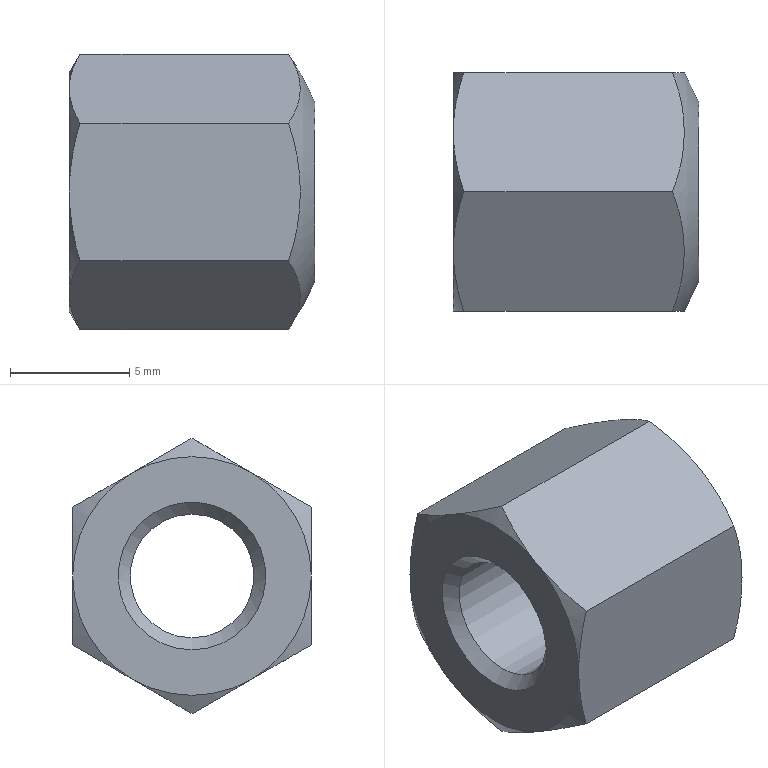Component | NX | GB804-1988_M6 | 1 solid | 18 faces | volume 652 mm3 | plane 8 | cone 8 | cylinder 1 | sphere 1 | commonest cylinder face diameters 5.188 x1